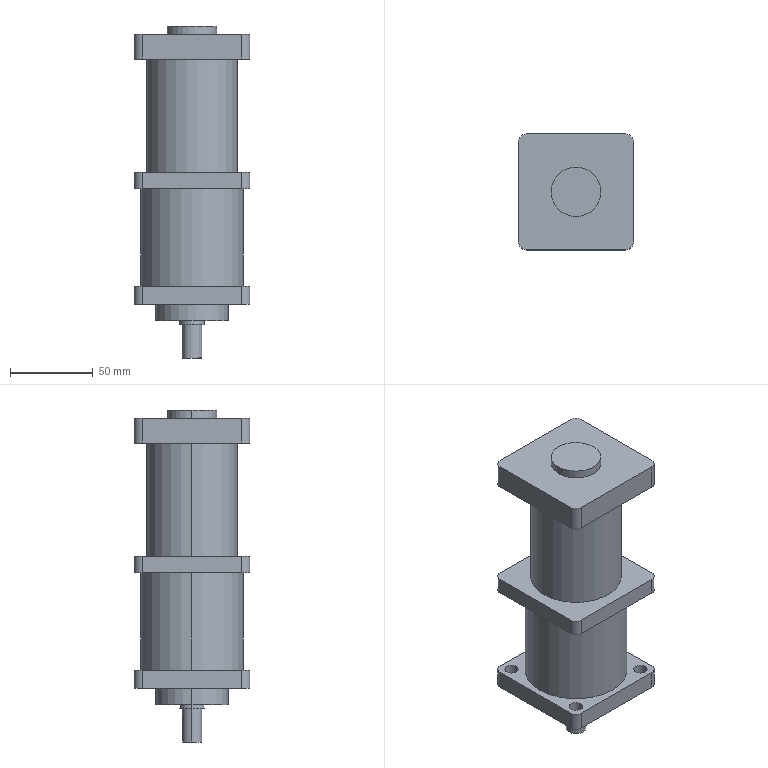Component | SolidWorks | GearedMotor-1 | 1 solid | 58 faces | box 70 x 70 x 201 mm | volume 535512 mm3 | cylinder 32 | plane 26 | commonest cylinder face diameters 10 x12 8 x8 30 x2 55 x2 62 x2 15 x2 44 x2 12 x2
build123d program:
from build123d import *

# Parameters (mm, degrees)
SKETCH1_W            = 70
SKETCH1_H            = 70
BOSS_EXTRUDE1_DEPTH  = 11
SKETCH2_R            = 22
BOSS_EXTRUDE2_DEPTH  = 10
SKETCH3_R            = 7.5
BOSS_EXTRUDE3_DEPTH  = 2.5
SKETCH4_R            = 6
BOSS_EXTRUDE5_DEPTH  = 20
CUT_EXTRUDE1_START   = 2.5
SKETCH6_W            = 4
SKETCH6_H            = 20.681
CUT_EXTRUDE1_DEPTH   = 5
SKETCH7_R            = 31
BOSS_EXTRUDE6_DEPTH  = 59
SKETCH8_W            = 70
SKETCH8_H            = 70
BOSS_EXTRUDE7_DEPTH  = 10
SKETCH9_R            = 27.5
BOSS_EXTRUDE8_DEPTH  = 68.5
SKETCH10_W           = 70
SKETCH10_H           = 70
BOSS_EXTRUDE9_DEPTH  = 15
SKETCH11_R           = 15
BOSS_EXTRUDE10_DEPTH = 5
FILLET2_R            = 5
CUT_EXTRUDE2_REACH   = 177.62
SKETCH13_R           = 4


with BuildPart() as part:
    # Sketch1 → Boss-Extrude1 (new body)
    with BuildSketch(Plane.XY):
        Rectangle(SKETCH1_W, SKETCH1_H)
    extrude(amount=BOSS_EXTRUDE1_DEPTH)

    # Sketch2 → Boss-Extrude2 (add)
    with BuildSketch(Plane.XY.offset(11)):
        with Locations(Location((0, 0, 0), (0, 0, 180))):
            Circle(SKETCH2_R)
    extrude(amount=BOSS_EXTRUDE2_DEPTH)

    # Sketch3 → Boss-Extrude3 (add)
    with BuildSketch(Plane.XY.offset(21)):
        Circle(SKETCH3_R)
    extrude(amount=BOSS_EXTRUDE3_DEPTH)

    # Sketch4 → Boss-Extrude5 (add)
    with BuildSketch(Plane.XY.offset(23.5)):
        Circle(SKETCH4_R)
    extrude(amount=BOSS_EXTRUDE5_DEPTH)

    # Sketch6 → Cut-Extrude1 (cut)
    with BuildSketch(Plane(origin=(0, 0, 0), x_dir=(1, 0, 0), z_dir=(0, 1, 0)).offset(CUT_EXTRUDE1_START)):
        with Locations((0, -37.84)):
            Rectangle(SKETCH6_W, SKETCH6_H)
    extrude(amount=CUT_EXTRUDE1_DEPTH, mode=Mode.SUBTRACT)

    # Sketch7 → Boss-Extrude6 (add)
    with BuildSketch(Plane(origin=(0, 0, 0), x_dir=(-1, 0, 0), z_dir=(0, 0, -1))):
        Circle(SKETCH7_R)
    extrude(amount=BOSS_EXTRUDE6_DEPTH)

    # Sketch8 → Boss-Extrude7 (add)
    with BuildSketch(Plane(origin=(0, 0, -59), x_dir=(-1, 0, 0), z_dir=(0, 0, -1))):
        Rectangle(SKETCH8_W, SKETCH8_H)
    extrude(amount=BOSS_EXTRUDE7_DEPTH)

    # Sketch9 → Boss-Extrude8 (add)
    with BuildSketch(Plane(origin=(0, 0, -69), x_dir=(-1, 0, 0), z_dir=(0, 0, -1))):
        with Locations(Location((0, 0, 0), (0, 0, 180))):
            Circle(SKETCH9_R)
    extrude(amount=BOSS_EXTRUDE8_DEPTH)

    # Sketch10 → Boss-Extrude9 (add)
    with BuildSketch(Plane(origin=(0, 0, -137.5), x_dir=(-1, 0, 0), z_dir=(0, 0, -1))):
        Rectangle(SKETCH10_W, SKETCH10_H)
    extrude(amount=BOSS_EXTRUDE9_DEPTH)

    # Sketch11 → Boss-Extrude10 (add)
    with BuildSketch(Plane(origin=(0, 0, -152.5), x_dir=(-1, 0, 0), z_dir=(0, 0, -1))):
        with Locations(Location((0, 0, 0), (0, 0, 180))):
            Circle(SKETCH11_R)
    extrude(amount=BOSS_EXTRUDE10_DEPTH)

    # Fillet2
    fillet2_edges = [part.edges().sort_by_distance(p)[0] for p in [
        (-35, -35, -64),
        (-35, 35, -64),
        (35, 35, -64),
        (35, -35, -64),
        (-35, -35, -145),
        (-35, 35, -145),
        (35, 35, -145),
        (35, -35, -145),
        (35, -35, 5.5),
        (-35, -35, 5.5),
        (-35, 35, 5.5),
        (35, 35, 5.5),
    ]]
    fillet(fillet2_edges, radius=FILLET2_R)

    # Sketch13 → Cut-Extrude2 (cut, up to next)
    with BuildSketch(Plane.XY.offset(11), mode=Mode.PRIVATE) as cut_extrude2_sk1:
        with Locations((-27.577, 27.577)):
            Circle(SKETCH13_R)
    cut_extrude2_tool1 = extrude(cut_extrude2_sk1.sketch, amount=-CUT_EXTRUDE2_REACH, mode=Mode.PRIVATE) & part.part
    # Sketch13 → Cut-Extrude2 (cut, up to next)
    with BuildSketch(Plane.XY.offset(11), mode=Mode.PRIVATE) as cut_extrude2_sk2:
        with Locations((27.577, 27.577)):
            Circle(SKETCH13_R)
    cut_extrude2_tool2 = extrude(cut_extrude2_sk2.sketch, amount=-CUT_EXTRUDE2_REACH, mode=Mode.PRIVATE) & part.part
    # Sketch13 → Cut-Extrude2 (cut, up to next)
    with BuildSketch(Plane.XY.offset(11), mode=Mode.PRIVATE) as cut_extrude2_sk3:
        with Locations((-27.577, -27.577)):
            Circle(SKETCH13_R)
    cut_extrude2_tool3 = extrude(cut_extrude2_sk3.sketch, amount=-CUT_EXTRUDE2_REACH, mode=Mode.PRIVATE) & part.part
    # Sketch13 → Cut-Extrude2 (cut, up to next)
    with BuildSketch(Plane.XY.offset(11), mode=Mode.PRIVATE) as cut_extrude2_sk4:
        with Locations((27.577, -27.577)):
            Circle(SKETCH13_R)
    cut_extrude2_tool4 = extrude(cut_extrude2_sk4.sketch, amount=-CUT_EXTRUDE2_REACH, mode=Mode.PRIVATE) & part.part
    add(cut_extrude2_tool1.solids().sort_by_distance((-27.577, 27.577, 11))[0], mode=Mode.SUBTRACT)
    add(cut_extrude2_tool2.solids().sort_by_distance((27.577, 27.577, 11))[0], mode=Mode.SUBTRACT)
    add(cut_extrude2_tool3.solids().sort_by_distance((-27.577, -27.577, 11))[0], mode=Mode.SUBTRACT)
    add(cut_extrude2_tool4.solids().sort_by_distance((27.577, -27.577, 11))[0], mode=Mode.SUBTRACT)


solid = part.part

# Placed as in the assembly
solid = solid.moved(Location((174.299, -234.1, 102.963), (-180, 0, 180)))